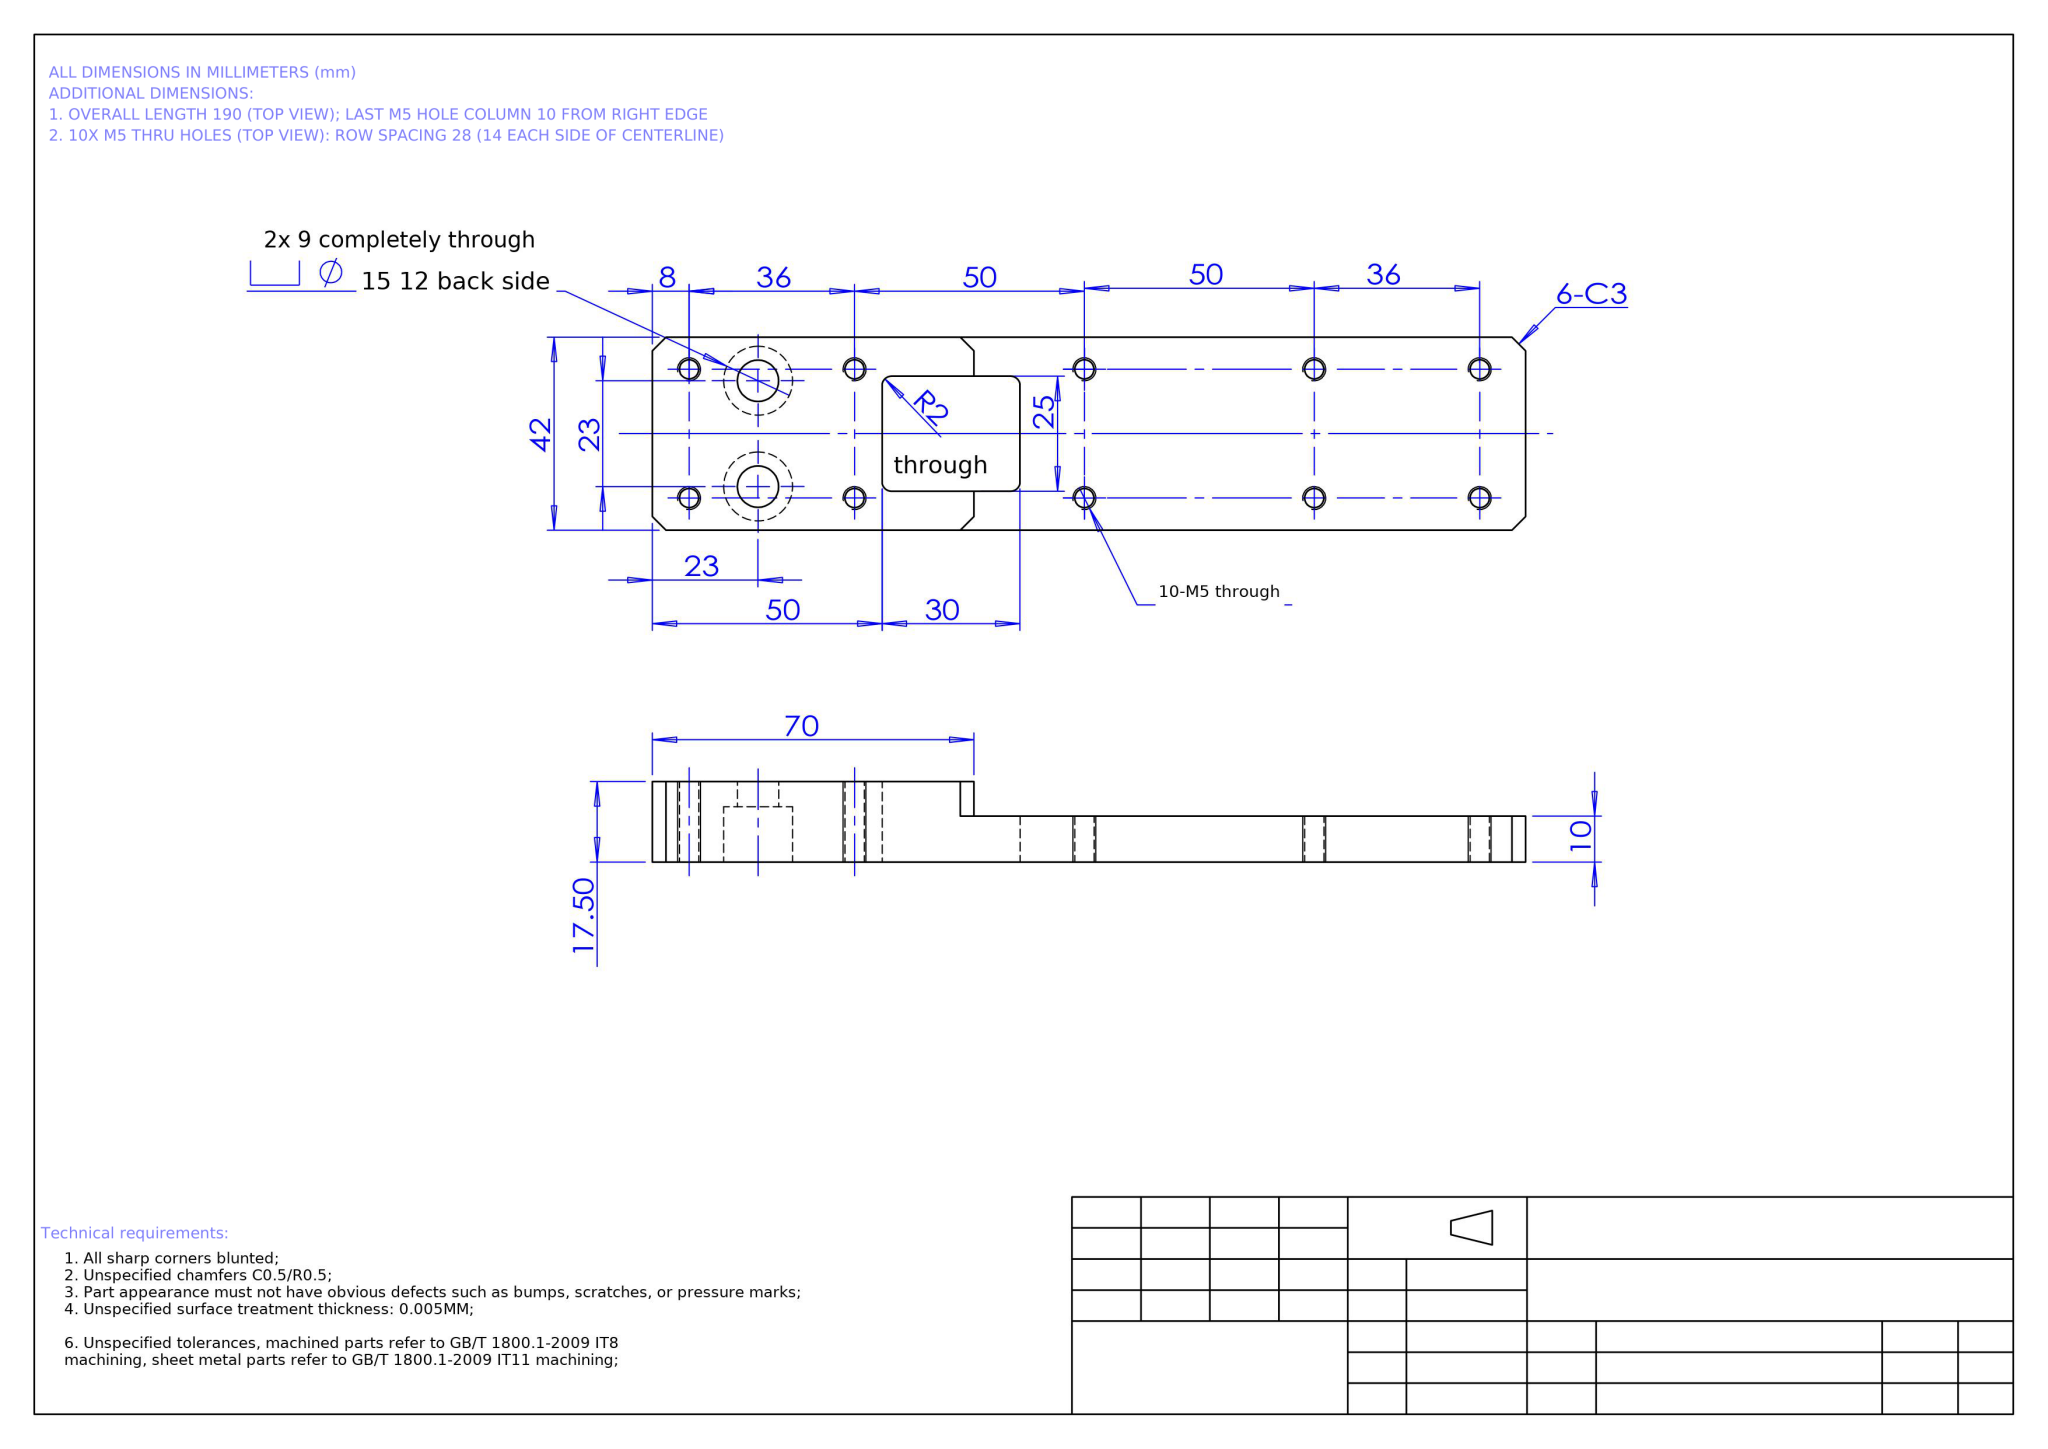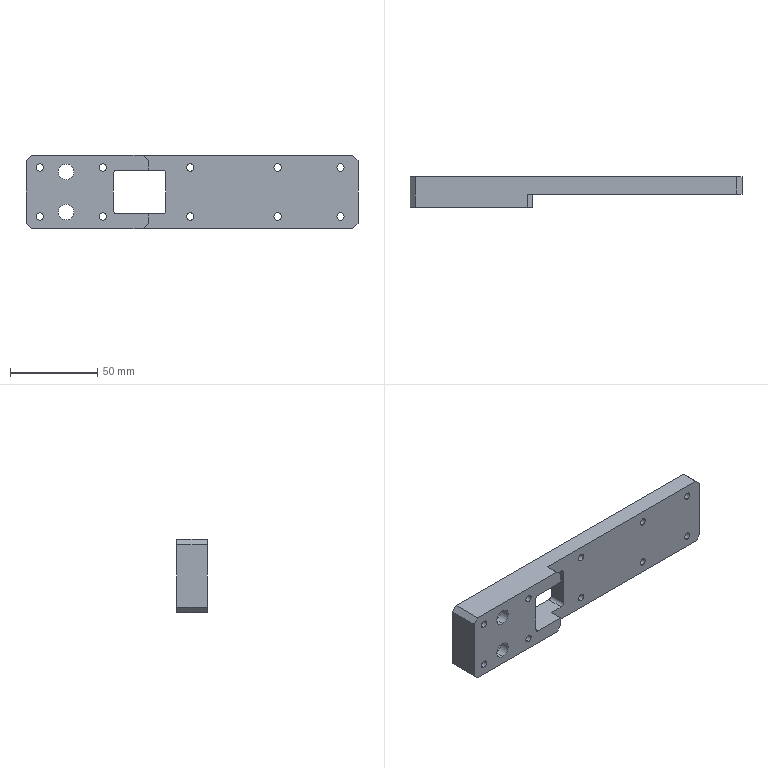Part | NX | mm | 1 solid | 53 faces | box 190 x 17.5 x 42 mm | volume 83590 mm3 | cylinder 32 | plane 21 | commonest cylinder face diameters 4.2 x20 15 x4 9 x4 4 x4